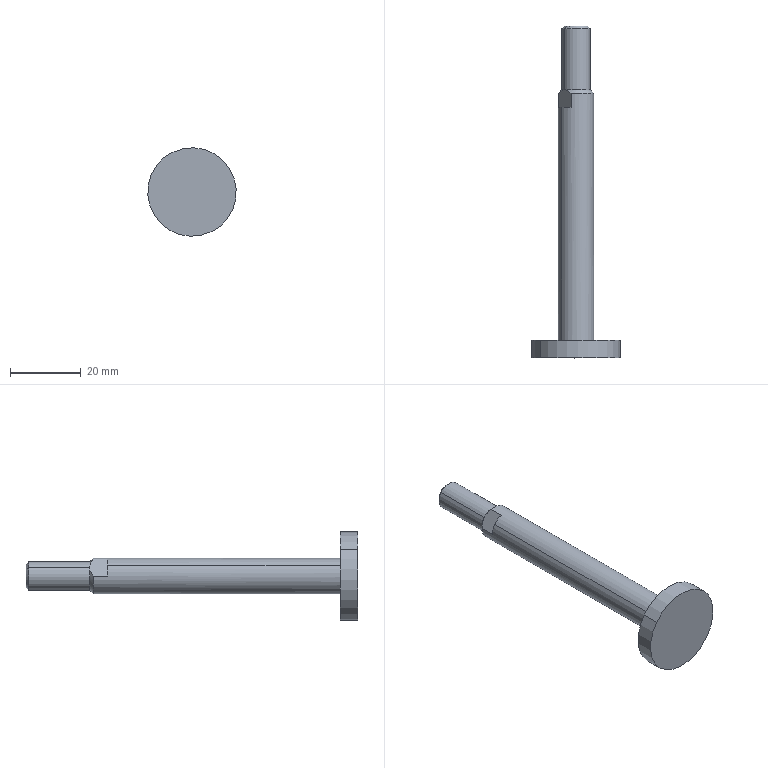Component | SolidWorks | HandlingMechanism-2_CDU25-40A-A93(0_0)-2_3..0..0.2-1 | 1 solid | 17 faces | box 25 x 93.75 x 25 mm | volume 8858 mm3 | plane 7 | cylinder 6 | cone 4 | commonest cylinder face diameters 10 x2 8 x2 25 x2
STEP:
#1=CARTESIAN_POINT('',(0.9638,4.508,6.134));
#2=VERTEX_POINT('',#1);
#3=CARTESIAN_POINT('',(0.8614,4.508,6.063));
#4=VERTEX_POINT('',#3);
#5=CARTESIAN_POINT('',(1.019,4.508,5.945));
#6=DIRECTION('',(0.,-1.,-0.));
#7=DIRECTION('',(0.8,0.,-0.6));
#8=AXIS2_PLACEMENT_3D('',#5,#6,#7);
#9=CIRCLE('',#8,0.1969);
#10=EDGE_CURVE('',#2,#4,#9,.T.);
#11=ORIENTED_EDGE('',*,*,#10,.T.);
#12=CARTESIAN_POINT('',(0.8614,1.919,6.063));
#13=VERTEX_POINT('',#12);
#14=CARTESIAN_POINT('',(0.8614,3.292,6.063));
#15=DIRECTION('',(0.,-1.,-0.));
#16=VECTOR('',#15,39.37);
#17=LINE('',#14,#16);
#18=EDGE_CURVE('',#4,#13,#17,.T.);
#19=ORIENTED_EDGE('',*,*,#18,.T.);
#20=CARTESIAN_POINT('',(1.176,1.919,5.827));
#21=VERTEX_POINT('',#20);
#22=CARTESIAN_POINT('',(1.019,1.919,5.945));
#23=DIRECTION('',(-0.,1.,0.));
#24=DIRECTION('',(0.8,0.,-0.6));
#25=AXIS2_PLACEMENT_3D('',#22,#23,#24);
#26=CIRCLE('',#25,0.1969);
#27=EDGE_CURVE('',#13,#21,#26,.T.);
#28=ORIENTED_EDGE('',*,*,#27,.T.);
#29=CARTESIAN_POINT('',(1.176,4.508,5.827));
#30=VERTEX_POINT('',#29);
#31=CARTESIAN_POINT('',(1.176,3.292,5.827));
#32=DIRECTION('',(0.,-1.,-0.));
#33=VECTOR('',#32,39.37);
#34=LINE('',#31,#33);
#35=EDGE_CURVE('',#30,#21,#34,.T.);
#36=ORIENTED_EDGE('',*,*,#35,.F.);
#37=CARTESIAN_POINT('',(1.216,4.508,5.945));
#38=VERTEX_POINT('',#37);
#39=CARTESIAN_POINT('',(1.019,4.508,5.945));
#40=DIRECTION('',(0.,-1.,-0.));
#41=DIRECTION('',(0.8,0.,-0.6));
#42=AXIS2_PLACEMENT_3D('',#39,#40,#41);
#43=CIRCLE('',#42,0.1969);
#44=EDGE_CURVE('',#30,#38,#43,.T.);
#45=ORIENTED_EDGE('',*,*,#44,.T.);
#46=CARTESIAN_POINT('',(1.216,4.665,5.945));
#47=VERTEX_POINT('',#46);
#48=CARTESIAN_POINT('',(1.216,3.292,5.945));
#49=DIRECTION('',(-0.,1.,0.));
#50=VECTOR('',#49,39.37);
#51=LINE('',#48,#50);
#52=EDGE_CURVE('',#38,#47,#51,.T.);
#53=ORIENTED_EDGE('',*,*,#52,.T.);
#54=CARTESIAN_POINT('',(0.9638,4.665,6.134));
#55=VERTEX_POINT('',#54);
#56=CARTESIAN_POINT('',(1.019,4.665,5.945));
#57=DIRECTION('',(0.,-1.,-0.));
#58=DIRECTION('',(0.8,0.,-0.6));
#59=AXIS2_PLACEMENT_3D('',#56,#57,#58);
#60=CIRCLE('',#59,0.1969);
#61=EDGE_CURVE('',#47,#55,#60,.T.);
#62=ORIENTED_EDGE('',*,*,#61,.T.);
#63=CARTESIAN_POINT('',(0.9638,3.292,6.134));
#64=DIRECTION('',(0.,-1.,-0.));
#65=VECTOR('',#64,39.37);
#66=LINE('',#63,#65);
#67=EDGE_CURVE('',#55,#2,#66,.T.);
#68=ORIENTED_EDGE('',*,*,#67,.T.);
#69=EDGE_LOOP('',(#11,#19,#28,#36,#45,#53,#62,#68));
#70=FACE_OUTER_BOUND('',#69,.T.);
#71=CARTESIAN_POINT('',(1.019,3.292,5.945));
#72=DIRECTION('',(0.,-1.,-0.));
#73=DIRECTION('',(0.8,0.,-0.6));
#74=AXIS2_PLACEMENT_3D('',#71,#72,#73);
#75=CYLINDRICAL_SURFACE('',#74,0.1969);
#76=ADVANCED_FACE('',(#70),#75,.T.);
#77=CARTESIAN_POINT('',(1.145,5.383,5.85));
#78=VERTEX_POINT('',#77);
#79=CARTESIAN_POINT('',(0.8929,5.383,6.039));
#80=VERTEX_POINT('',#79);
#81=CARTESIAN_POINT('',(1.019,5.383,5.945));
#82=DIRECTION('',(0.,-1.,-0.));
#83=DIRECTION('',(0.8,0.,-0.6));
#84=AXIS2_PLACEMENT_3D('',#81,#82,#83);
#85=CIRCLE('',#84,0.1575);
#86=EDGE_CURVE('',#78,#80,#85,.T.);
#87=ORIENTED_EDGE('',*,*,#86,.T.);
#88=CARTESIAN_POINT('',(0.8929,4.705,6.039));
#89=VERTEX_POINT('',#88);
#90=CARTESIAN_POINT('',(0.8929,5.044,6.039));
#91=DIRECTION('',(0.,-1.,-0.));
#92=VECTOR('',#91,39.37);
#93=LINE('',#90,#92);
#94=EDGE_CURVE('',#80,#89,#93,.T.);
#95=ORIENTED_EDGE('',*,*,#94,.T.);
#96=CARTESIAN_POINT('',(1.145,4.705,5.85));
#97=VERTEX_POINT('',#96);
#98=CARTESIAN_POINT('',(1.019,4.705,5.945));
#99=DIRECTION('',(0.,-1.,-0.));
#100=DIRECTION('',(0.6,0.,0.8));
#101=AXIS2_PLACEMENT_3D('',#98,#99,#100);
#102=CIRCLE('',#101,0.1575);
#103=EDGE_CURVE('',#97,#89,#102,.T.);
#104=ORIENTED_EDGE('',*,*,#103,.F.);
#105=CARTESIAN_POINT('',(1.145,5.044,5.85));
#106=DIRECTION('',(0.,-1.,-0.));
#107=VECTOR('',#106,39.37);
#108=LINE('',#105,#107);
#109=EDGE_CURVE('',#78,#97,#108,.T.);
#110=ORIENTED_EDGE('',*,*,#109,.F.);
#111=EDGE_LOOP('',(#87,#95,#104,#110));
#112=FACE_OUTER_BOUND('',#111,.T.);
#113=CARTESIAN_POINT('',(1.019,5.044,5.945));
#114=DIRECTION('',(0.,-1.,-0.));
#115=DIRECTION('',(0.8,0.,-0.6));
#116=AXIS2_PLACEMENT_3D('',#113,#114,#115);
#117=CYLINDRICAL_SURFACE('',#116,0.1575);
#118=ADVANCED_FACE('',(#112),#117,.T.);
#119=CARTESIAN_POINT('',(0.6252,1.919,6.24));
#120=VERTEX_POINT('',#119);
#121=CARTESIAN_POINT('',(1.413,1.919,5.65));
#122=VERTEX_POINT('',#121);
#123=CARTESIAN_POINT('',(1.019,1.919,5.945));
#124=DIRECTION('',(-0.,1.,0.));
#125=DIRECTION('',(0.8,0.,-0.6));
#126=AXIS2_PLACEMENT_3D('',#123,#124,#125);
#127=CIRCLE('',#126,0.4921);
#128=EDGE_CURVE('',#120,#122,#127,.T.);
#129=ORIENTED_EDGE('',*,*,#128,.F.);
#130=CARTESIAN_POINT('',(0.6252,1.722,6.24));
#131=VERTEX_POINT('',#130);
#132=CARTESIAN_POINT('',(0.6252,1.821,6.24));
#133=DIRECTION('',(0.,-1.,-0.));
#134=VECTOR('',#133,39.37);
#135=LINE('',#132,#134);
#136=EDGE_CURVE('',#120,#131,#135,.T.);
#137=ORIENTED_EDGE('',*,*,#136,.T.);
#138=CARTESIAN_POINT('',(1.413,1.722,5.65));
#139=VERTEX_POINT('',#138);
#140=CARTESIAN_POINT('',(1.019,1.722,5.945));
#141=DIRECTION('',(-0.,1.,0.));
#142=DIRECTION('',(0.8,0.,-0.6));
#143=AXIS2_PLACEMENT_3D('',#140,#141,#142);
#144=CIRCLE('',#143,0.4921);
#145=EDGE_CURVE('',#131,#139,#144,.T.);
#146=ORIENTED_EDGE('',*,*,#145,.T.);
#147=CARTESIAN_POINT('',(1.413,1.821,5.65));
#148=DIRECTION('',(0.,-1.,-0.));
#149=VECTOR('',#148,39.37);
#150=LINE('',#147,#149);
#151=EDGE_CURVE('',#122,#139,#150,.T.);
#152=ORIENTED_EDGE('',*,*,#151,.F.);
#153=EDGE_LOOP('',(#129,#137,#146,#152));
#154=FACE_OUTER_BOUND('',#153,.T.);
#155=CARTESIAN_POINT('',(1.019,1.821,5.945));
#156=DIRECTION('',(0.,-1.,-0.));
#157=DIRECTION('',(0.8,0.,-0.6));
#158=AXIS2_PLACEMENT_3D('',#155,#156,#157);
#159=CYLINDRICAL_SURFACE('',#158,0.4921);
#160=ADVANCED_FACE('',(#154),#159,.T.);
#161=CARTESIAN_POINT('',(1.121,5.413,5.869));
#162=VERTEX_POINT('',#161);
#163=CARTESIAN_POINT('',(0.9171,5.413,6.021));
#164=VERTEX_POINT('',#163);
#165=CARTESIAN_POINT('',(1.019,5.413,5.945));
#166=DIRECTION('',(0.,-1.,-0.));
#167=DIRECTION('',(0.8,0.,-0.6));
#168=AXIS2_PLACEMENT_3D('',#165,#166,#167);
#169=CIRCLE('',#168,0.1273);
#170=EDGE_CURVE('',#162,#164,#169,.T.);
#171=ORIENTED_EDGE('',*,*,#170,.T.);
#172=CARTESIAN_POINT('',(0.8929,5.383,6.039));
#173=DIRECTION('',(-0.5657,-0.7071,0.4243));
#174=VECTOR('',#173,39.37);
#175=LINE('',#172,#174);
#176=EDGE_CURVE('',#164,#80,#175,.T.);
#177=ORIENTED_EDGE('',*,*,#176,.T.);
#178=ORIENTED_EDGE('',*,*,#86,.F.);
#179=CARTESIAN_POINT('',(1.145,5.383,5.85));
#180=DIRECTION('',(0.5657,-0.7071,-0.4243));
#181=VECTOR('',#180,39.37);
#182=LINE('',#179,#181);
#183=EDGE_CURVE('',#162,#78,#182,.T.);
#184=ORIENTED_EDGE('',*,*,#183,.F.);
#185=EDGE_LOOP('',(#171,#177,#178,#184));
#186=FACE_OUTER_BOUND('',#185,.T.);
#187=CARTESIAN_POINT('',(1.019,5.383,5.945));
#188=DIRECTION('',(0.,-1.,-0.));
#189=DIRECTION('',(0.8,0.,-0.6));
#190=AXIS2_PLACEMENT_3D('',#187,#188,#189);
#191=CONICAL_SURFACE('',#190,0.1575,0.7854);
#192=ADVANCED_FACE('',(#186),#191,.T.);
#193=ORIENTED_EDGE('',*,*,#18,.F.);
#194=CARTESIAN_POINT('',(0.8221,4.508,5.945));
#195=VERTEX_POINT('',#194);
#196=CARTESIAN_POINT('',(1.019,4.508,5.945));
#197=DIRECTION('',(0.,-1.,-0.));
#198=DIRECTION('',(0.8,0.,-0.6));
#199=AXIS2_PLACEMENT_3D('',#196,#197,#198);
#200=CIRCLE('',#199,0.1969);
#201=EDGE_CURVE('',#4,#195,#200,.T.);
#202=ORIENTED_EDGE('',*,*,#201,.T.);
#203=CARTESIAN_POINT('',(0.8221,4.665,5.945));
#204=VERTEX_POINT('',#203);
#205=CARTESIAN_POINT('',(0.8221,3.292,5.945));
#206=DIRECTION('',(-0.,1.,0.));
#207=VECTOR('',#206,39.37);
#208=LINE('',#205,#207);
#209=EDGE_CURVE('',#195,#204,#208,.T.);
#210=ORIENTED_EDGE('',*,*,#209,.T.);
#211=CARTESIAN_POINT('',(1.074,4.665,5.756));
#212=VERTEX_POINT('',#211);
#213=CARTESIAN_POINT('',(1.019,4.665,5.945));
#214=DIRECTION('',(0.,-1.,-0.));
#215=DIRECTION('',(0.8,0.,-0.6));
#216=AXIS2_PLACEMENT_3D('',#213,#214,#215);
#217=CIRCLE('',#216,0.1969);
#218=EDGE_CURVE('',#204,#212,#217,.T.);
#219=ORIENTED_EDGE('',*,*,#218,.T.);
#220=CARTESIAN_POINT('',(1.074,4.508,5.756));
#221=VERTEX_POINT('',#220);
#222=CARTESIAN_POINT('',(1.074,3.292,5.756));
#223=DIRECTION('',(0.,-1.,-0.));
#224=VECTOR('',#223,39.37);
#225=LINE('',#222,#224);
#226=EDGE_CURVE('',#212,#221,#225,.T.);
#227=ORIENTED_EDGE('',*,*,#226,.T.);
#228=CARTESIAN_POINT('',(1.019,4.508,5.945));
#229=DIRECTION('',(0.,-1.,-0.));
#230=DIRECTION('',(0.8,0.,-0.6));
#231=AXIS2_PLACEMENT_3D('',#228,#229,#230);
#232=CIRCLE('',#231,0.1969);
#233=EDGE_CURVE('',#221,#30,#232,.T.);
#234=ORIENTED_EDGE('',*,*,#233,.T.);
#235=ORIENTED_EDGE('',*,*,#35,.T.);
#236=CARTESIAN_POINT('',(1.019,1.919,5.945));
#237=DIRECTION('',(-0.,1.,0.));
#238=DIRECTION('',(0.8,0.,-0.6));
#239=AXIS2_PLACEMENT_3D('',#236,#237,#238);
#240=CIRCLE('',#239,0.1969);
#241=EDGE_CURVE('',#21,#13,#240,.T.);
#242=ORIENTED_EDGE('',*,*,#241,.T.);
#243=EDGE_LOOP('',(#193,#202,#210,#219,#227,#234,#235,#242));
#244=FACE_OUTER_BOUND('',#243,.T.);
#245=CARTESIAN_POINT('',(1.019,3.292,5.945));
#246=DIRECTION('',(0.,-1.,-0.));
#247=DIRECTION('',(0.8,0.,-0.6));
#248=AXIS2_PLACEMENT_3D('',#245,#246,#247);
#249=CYLINDRICAL_SURFACE('',#248,0.1969);
#250=ADVANCED_FACE('',(#244),#249,.T.);
#251=CARTESIAN_POINT('',(1.216,4.665,5.945));
#252=CARTESIAN_POINT('',(1.205,4.676,5.93));
#253=CARTESIAN_POINT('',(1.194,4.686,5.916));
#254=CARTESIAN_POINT('',(1.176,4.697,5.892));
#255=CARTESIAN_POINT('',(1.17,4.7,5.884));
#256=CARTESIAN_POINT('',(1.158,4.704,5.867));
#257=CARTESIAN_POINT('',(1.151,4.705,5.859));
#258=CARTESIAN_POINT('',(1.145,4.705,5.85));
#259=B_SPLINE_CURVE_WITH_KNOTS('',3,(#251,#252,#253,#254,#255,#256,#257,#258),.UNSPECIFIED.,.F.,.F.,(4,2,2,4),(0.,0.001595,0.002392,0.003189),.UNSPECIFIED.);
#260=EDGE_CURVE('',#47,#97,#259,.T.);
#261=ORIENTED_EDGE('',*,*,#260,.T.);
#262=ORIENTED_EDGE('',*,*,#103,.T.);
#263=CARTESIAN_POINT('',(0.8929,4.705,6.039));
#264=CARTESIAN_POINT('',(0.8993,4.705,6.048));
#265=CARTESIAN_POINT('',(0.9055,4.704,6.056));
#266=CARTESIAN_POINT('',(0.9179,4.7,6.073));
#267=CARTESIAN_POINT('',(0.9239,4.697,6.081));
#268=CARTESIAN_POINT('',(0.9418,4.686,6.104));
#269=CARTESIAN_POINT('',(0.953,4.676,6.119));
#270=CARTESIAN_POINT('',(0.9638,4.665,6.134));
#271=B_SPLINE_CURVE_WITH_KNOTS('',3,(#263,#264,#265,#266,#267,#268,#269,#270),.UNSPECIFIED.,.F.,.F.,(4,2,2,4),(0.,0.0007961,0.001592,0.003185),.UNSPECIFIED.);
#272=EDGE_CURVE('',#89,#55,#271,.T.);
#273=ORIENTED_EDGE('',*,*,#272,.T.);
#274=ORIENTED_EDGE('',*,*,#61,.F.);
#275=EDGE_LOOP('',(#261,#262,#273,#274));
#276=FACE_OUTER_BOUND('',#275,.T.);
#277=CARTESIAN_POINT('',(1.019,4.665,5.945));
#278=DIRECTION('',(0.,-1.,-0.));
#279=DIRECTION('',(0.8,0.,-0.6));
#280=AXIS2_PLACEMENT_3D('',#277,#278,#279);
#281=CONICAL_SURFACE('',#280,0.1969,0.7854);
#282=ADVANCED_FACE('',(#276),#281,.T.);
#283=ORIENTED_EDGE('',*,*,#260,.F.);
#284=ORIENTED_EDGE('',*,*,#52,.F.);
#285=CARTESIAN_POINT('',(1.216,4.508,5.945));
#286=DIRECTION('',(0.6,0.,0.8));
#287=VECTOR('',#286,39.37);
#288=LINE('',#285,#287);
#289=EDGE_CURVE('',#221,#38,#288,.T.);
#290=ORIENTED_EDGE('',*,*,#289,.F.);
#291=ORIENTED_EDGE('',*,*,#226,.F.);
#292=CARTESIAN_POINT('',(1.145,4.705,5.85));
#293=CARTESIAN_POINT('',(1.139,4.705,5.842));
#294=CARTESIAN_POINT('',(1.132,4.704,5.834));
#295=CARTESIAN_POINT('',(1.12,4.7,5.817));
#296=CARTESIAN_POINT('',(1.114,4.697,5.809));
#297=CARTESIAN_POINT('',(1.096,4.686,5.785));
#298=CARTESIAN_POINT('',(1.085,4.676,5.77));
#299=CARTESIAN_POINT('',(1.074,4.665,5.756));
#300=B_SPLINE_CURVE_WITH_KNOTS('',3,(#292,#293,#294,#295,#296,#297,#298,#299),.UNSPECIFIED.,.F.,.F.,(4,2,2,4),(0.,0.0007961,0.001592,0.003185),.UNSPECIFIED.);
#301=EDGE_CURVE('',#97,#212,#300,.T.);
#302=ORIENTED_EDGE('',*,*,#301,.F.);
#303=EDGE_LOOP('',(#283,#284,#290,#291,#302));
#304=FACE_OUTER_BOUND('',#303,.T.);
#305=CARTESIAN_POINT('',(1.216,4.508,5.945));
#306=DIRECTION('',(-0.8,-0.,0.6));
#307=DIRECTION('',(0.,-1.,-0.));
#308=AXIS2_PLACEMENT_3D('',#305,#306,#307);
#309=PLANE('',#308);
#310=ADVANCED_FACE('',(#304),#309,.F.);
#311=ORIENTED_EDGE('',*,*,#233,.F.);
#312=ORIENTED_EDGE('',*,*,#289,.T.);
#313=ORIENTED_EDGE('',*,*,#44,.F.);
#314=EDGE_LOOP('',(#311,#312,#313));
#315=FACE_OUTER_BOUND('',#314,.T.);
#316=CARTESIAN_POINT('',(1.019,4.508,5.945));
#317=DIRECTION('',(-0.,1.,0.));
#318=DIRECTION('',(-0.8,-0.,0.6));
#319=AXIS2_PLACEMENT_3D('',#316,#317,#318);
#320=PLANE('',#319);
#321=ADVANCED_FACE('',(#315),#320,.T.);
#322=ORIENTED_EDGE('',*,*,#301,.T.);
#323=ORIENTED_EDGE('',*,*,#218,.F.);
#324=CARTESIAN_POINT('',(0.8221,4.665,5.945));
#325=CARTESIAN_POINT('',(0.8329,4.676,5.959));
#326=CARTESIAN_POINT('',(0.8441,4.686,5.974));
#327=CARTESIAN_POINT('',(0.8618,4.697,5.998));
#328=CARTESIAN_POINT('',(0.8679,4.7,6.006));
#329=CARTESIAN_POINT('',(0.8803,4.704,6.023));
#330=CARTESIAN_POINT('',(0.8866,4.705,6.031));
#331=CARTESIAN_POINT('',(0.8929,4.705,6.039));
#332=B_SPLINE_CURVE_WITH_KNOTS('',3,(#324,#325,#326,#327,#328,#329,#330,#331),.UNSPECIFIED.,.F.,.F.,(4,2,2,4),(0.,0.001595,0.002392,0.003189),.UNSPECIFIED.);
#333=EDGE_CURVE('',#204,#89,#332,.T.);
#334=ORIENTED_EDGE('',*,*,#333,.T.);
#335=CARTESIAN_POINT('',(1.019,4.705,5.945));
#336=DIRECTION('',(0.,-1.,-0.));
#337=DIRECTION('',(0.6,0.,0.8));
#338=AXIS2_PLACEMENT_3D('',#335,#336,#337);
#339=CIRCLE('',#338,0.1575);
#340=EDGE_CURVE('',#89,#97,#339,.T.);
#341=ORIENTED_EDGE('',*,*,#340,.T.);
#342=EDGE_LOOP('',(#322,#323,#334,#341));
#343=FACE_OUTER_BOUND('',#342,.T.);
#344=CARTESIAN_POINT('',(1.019,4.665,5.945));
#345=DIRECTION('',(0.,-1.,-0.));
#346=DIRECTION('',(0.8,0.,-0.6));
#347=AXIS2_PLACEMENT_3D('',#344,#345,#346);
#348=CONICAL_SURFACE('',#347,0.1969,0.7854);
#349=ADVANCED_FACE('',(#343),#348,.T.);
#350=CARTESIAN_POINT('',(1.019,1.919,5.945));
#351=DIRECTION('',(-0.,1.,0.));
#352=DIRECTION('',(0.8,0.,-0.6));
#353=AXIS2_PLACEMENT_3D('',#350,#351,#352);
#354=CIRCLE('',#353,0.4921);
#355=EDGE_CURVE('',#122,#120,#354,.T.);
#356=ORIENTED_EDGE('',*,*,#355,.T.);
#357=ORIENTED_EDGE('',*,*,#128,.T.);
#358=EDGE_LOOP('',(#356,#357));
#359=FACE_OUTER_BOUND('',#358,.T.);
#360=ORIENTED_EDGE('',*,*,#241,.F.);
#361=ORIENTED_EDGE('',*,*,#27,.F.);
#362=EDGE_LOOP('',(#360,#361));
#363=FACE_BOUND('',#362,.T.);
#364=CARTESIAN_POINT('',(1.226,1.919,6.22));
#365=DIRECTION('',(-0.,1.,0.));
#366=DIRECTION('',(-0.8,-0.,0.6));
#367=AXIS2_PLACEMENT_3D('',#364,#365,#366);
#368=PLANE('',#367);
#369=ADVANCED_FACE('',(#359,#363),#368,.T.);
#370=ORIENTED_EDGE('',*,*,#94,.F.);
#371=CARTESIAN_POINT('',(1.019,5.383,5.945));
#372=DIRECTION('',(0.,-1.,-0.));
#373=DIRECTION('',(0.8,0.,-0.6));
#374=AXIS2_PLACEMENT_3D('',#371,#372,#373);
#375=CIRCLE('',#374,0.1575);
#376=EDGE_CURVE('',#80,#78,#375,.T.);
#377=ORIENTED_EDGE('',*,*,#376,.T.);
#378=ORIENTED_EDGE('',*,*,#109,.T.);
#379=ORIENTED_EDGE('',*,*,#340,.F.);
#380=EDGE_LOOP('',(#370,#377,#378,#379));
#381=FACE_OUTER_BOUND('',#380,.T.);
#382=CARTESIAN_POINT('',(1.019,5.044,5.945));
#383=DIRECTION('',(0.,-1.,-0.));
#384=DIRECTION('',(0.8,0.,-0.6));
#385=AXIS2_PLACEMENT_3D('',#382,#383,#384);
#386=CYLINDRICAL_SURFACE('',#385,0.1575);
#387=ADVANCED_FACE('',(#381),#386,.T.);
#388=ORIENTED_EDGE('',*,*,#209,.F.);
#389=CARTESIAN_POINT('',(0.8221,4.508,5.945));
#390=DIRECTION('',(-0.6,-0.,-0.8));
#391=VECTOR('',#390,39.37);
#392=LINE('',#389,#391);
#393=EDGE_CURVE('',#2,#195,#392,.T.);
#394=ORIENTED_EDGE('',*,*,#393,.F.);
#395=ORIENTED_EDGE('',*,*,#67,.F.);
#396=ORIENTED_EDGE('',*,*,#272,.F.);
#397=ORIENTED_EDGE('',*,*,#333,.F.);
#398=EDGE_LOOP('',(#388,#394,#395,#396,#397));
#399=FACE_OUTER_BOUND('',#398,.T.);
#400=CARTESIAN_POINT('',(0.8221,4.508,5.945));
#401=DIRECTION('',(0.8,0.,-0.6));
#402=DIRECTION('',(-0.,1.,0.));
#403=AXIS2_PLACEMENT_3D('',#400,#401,#402);
#404=PLANE('',#403);
#405=ADVANCED_FACE('',(#399),#404,.F.);
#406=ORIENTED_EDGE('',*,*,#10,.F.);
#407=ORIENTED_EDGE('',*,*,#393,.T.);
#408=ORIENTED_EDGE('',*,*,#201,.F.);
#409=EDGE_LOOP('',(#406,#407,#408));
#410=FACE_OUTER_BOUND('',#409,.T.);
#411=CARTESIAN_POINT('',(1.019,4.508,5.945));
#412=DIRECTION('',(-0.,1.,0.));
#413=DIRECTION('',(-0.8,-0.,0.6));
#414=AXIS2_PLACEMENT_3D('',#411,#412,#413);
#415=PLANE('',#414);
#416=ADVANCED_FACE('',(#410),#415,.T.);
#417=ORIENTED_EDGE('',*,*,#136,.F.);
#418=ORIENTED_EDGE('',*,*,#355,.F.);
#419=ORIENTED_EDGE('',*,*,#151,.T.);
#420=CARTESIAN_POINT('',(1.019,1.722,5.945));
#421=DIRECTION('',(-0.,1.,0.));
#422=DIRECTION('',(0.8,0.,-0.6));
#423=AXIS2_PLACEMENT_3D('',#420,#421,#422);
#424=CIRCLE('',#423,0.4921);
#425=EDGE_CURVE('',#139,#131,#424,.T.);
#426=ORIENTED_EDGE('',*,*,#425,.T.);
#427=EDGE_LOOP('',(#417,#418,#419,#426));
#428=FACE_OUTER_BOUND('',#427,.T.);
#429=CARTESIAN_POINT('',(1.019,1.821,5.945));
#430=DIRECTION('',(0.,-1.,-0.));
#431=DIRECTION('',(0.8,0.,-0.6));
#432=AXIS2_PLACEMENT_3D('',#429,#430,#431);
#433=CYLINDRICAL_SURFACE('',#432,0.4921);
#434=ADVANCED_FACE('',(#428),#433,.T.);
#435=ORIENTED_EDGE('',*,*,#176,.F.);
#436=CARTESIAN_POINT('',(1.019,5.413,5.945));
#437=DIRECTION('',(0.,-1.,-0.));
#438=DIRECTION('',(0.8,0.,-0.6));
#439=AXIS2_PLACEMENT_3D('',#436,#437,#438);
#440=CIRCLE('',#439,0.1273);
#441=EDGE_CURVE('',#164,#162,#440,.T.);
#442=ORIENTED_EDGE('',*,*,#441,.T.);
#443=ORIENTED_EDGE('',*,*,#183,.T.);
#444=ORIENTED_EDGE('',*,*,#376,.F.);
#445=EDGE_LOOP('',(#435,#442,#443,#444));
#446=FACE_OUTER_BOUND('',#445,.T.);
#447=CARTESIAN_POINT('',(1.019,5.383,5.945));
#448=DIRECTION('',(0.,-1.,-0.));
#449=DIRECTION('',(0.8,0.,-0.6));
#450=AXIS2_PLACEMENT_3D('',#447,#448,#449);
#451=CONICAL_SURFACE('',#450,0.1575,0.7854);
#452=ADVANCED_FACE('',(#446),#451,.T.);
#453=ORIENTED_EDGE('',*,*,#425,.F.);
#454=ORIENTED_EDGE('',*,*,#145,.F.);
#455=EDGE_LOOP('',(#453,#454));
#456=FACE_OUTER_BOUND('',#455,.T.);
#457=CARTESIAN_POINT('',(1.167,1.722,6.142));
#458=DIRECTION('',(0.,-1.,-0.));
#459=DIRECTION('',(0.8,0.,-0.6));
#460=AXIS2_PLACEMENT_3D('',#457,#458,#459);
#461=PLANE('',#460);
#462=ADVANCED_FACE('',(#456),#461,.T.);
#463=ORIENTED_EDGE('',*,*,#170,.F.);
#464=ORIENTED_EDGE('',*,*,#441,.F.);
#465=EDGE_LOOP('',(#463,#464));
#466=FACE_OUTER_BOUND('',#465,.T.);
#467=CARTESIAN_POINT('',(1.057,5.413,5.996));
#468=DIRECTION('',(-0.,1.,0.));
#469=DIRECTION('',(-0.8,-0.,0.6));
#470=AXIS2_PLACEMENT_3D('',#467,#468,#469);
#471=PLANE('',#470);
#472=ADVANCED_FACE('',(#466),#471,.T.);
#473=CLOSED_SHELL('',(#76,#118,#160,#192,#250,#282,#310,#321,#349,#369,#387,#405,#416,#434,#452,#462,#472));
#474=MANIFOLD_SOLID_BREP('',#473);
#475=CARTESIAN_POINT('',(0.,0.,0.));
#476=DIRECTION('',(0.,0.,1.));
#477=DIRECTION('',(1.,0.,0.));
#478=AXIS2_PLACEMENT_3D('',#475,#476,#477);
#479=(LENGTH_UNIT()NAMED_UNIT(*)SI_UNIT($,.METRE.));
#480=LENGTH_MEASURE_WITH_UNIT(LENGTH_MEASURE(0.0254),#479);
#481=DIMENSIONAL_EXPONENTS(1.,0.,0.,0.,0.,0.,0.);
#482=(CONVERSION_BASED_UNIT('',#480)LENGTH_UNIT()NAMED_UNIT(#481));
#483=UNCERTAINTY_MEASURE_WITH_UNIT(LENGTH_MEASURE(0.00001),#482,'','');
#484=(NAMED_UNIT(*)PLANE_ANGLE_UNIT()SI_UNIT($,.RADIAN.));
#485=(NAMED_UNIT(*)SI_UNIT($,.STERADIAN.)SOLID_ANGLE_UNIT());
#486=(GEOMETRIC_REPRESENTATION_CONTEXT(3)GLOBAL_UNCERTAINTY_ASSIGNED_CONTEXT((#483))GLOBAL_UNIT_ASSIGNED_CONTEXT((#482,#484,#485))REPRESENTATION_CONTEXT('',''));
#487=ADVANCED_BREP_SHAPE_REPRESENTATION('',(#474,#478),#486);
#488=COLOUR_RGB('',0.7922,0.8196,0.9333);
#489=FILL_AREA_STYLE_COLOUR('',#488);
#490=FILL_AREA_STYLE('',(#489));
#491=SURFACE_STYLE_FILL_AREA(#490);
#492=SURFACE_SIDE_STYLE('',(#491));
#493=SURFACE_STYLE_USAGE(.BOTH.,#492);
#494=PRESENTATION_STYLE_ASSIGNMENT((#493));
#495=STYLED_ITEM('',(#494),#474);
#496=(LENGTH_UNIT()NAMED_UNIT(*)SI_UNIT($,.METRE.));
#497=LENGTH_MEASURE_WITH_UNIT(LENGTH_MEASURE(0.0254),#496);
#498=DIMENSIONAL_EXPONENTS(1.,0.,0.,0.,0.,0.,0.);
#499=(CONVERSION_BASED_UNIT('',#497)LENGTH_UNIT()NAMED_UNIT(#498));
#500=UNCERTAINTY_MEASURE_WITH_UNIT(LENGTH_MEASURE(0.00001),#499,'','');
#501=(NAMED_UNIT(*)PLANE_ANGLE_UNIT()SI_UNIT($,.RADIAN.));
#502=(NAMED_UNIT(*)SI_UNIT($,.STERADIAN.)SOLID_ANGLE_UNIT());
#503=(GEOMETRIC_REPRESENTATION_CONTEXT(3)GLOBAL_UNCERTAINTY_ASSIGNED_CONTEXT((#500))GLOBAL_UNIT_ASSIGNED_CONTEXT((#499,#501,#502))REPRESENTATION_CONTEXT('',''));
#504=MECHANICAL_DESIGN_GEOMETRIC_PRESENTATION_REPRESENTATION('',(#495),#503);
#505=PRESENTATION_LAYER_ASSIGNMENT('','',(#495));